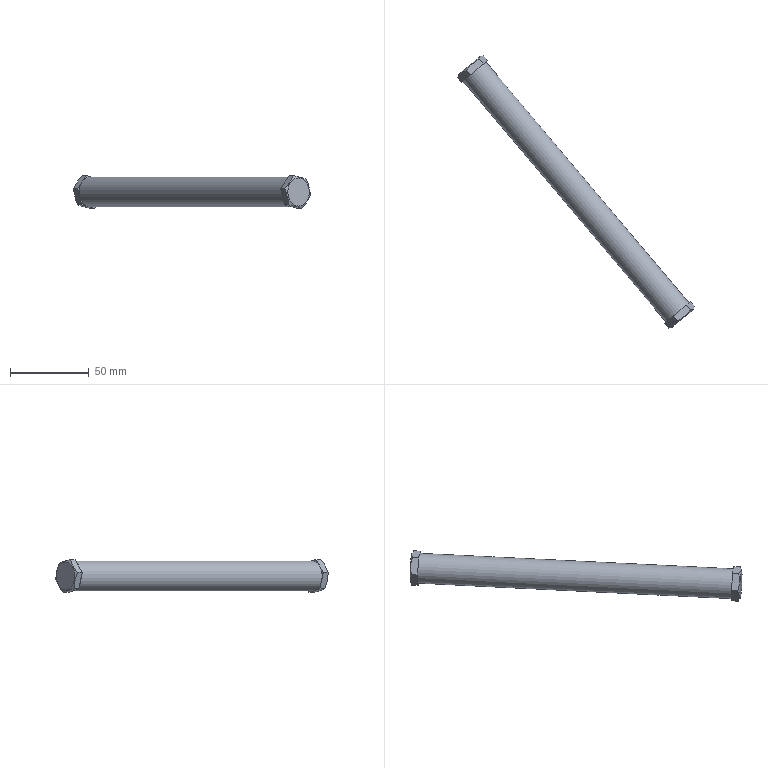Component | NX | PERNO4 | 1 solid | 29 faces | volume 59798 mm3 | plane 26 | cone 2 | cylinder 1 | commonest cylinder face diameters 19 x1